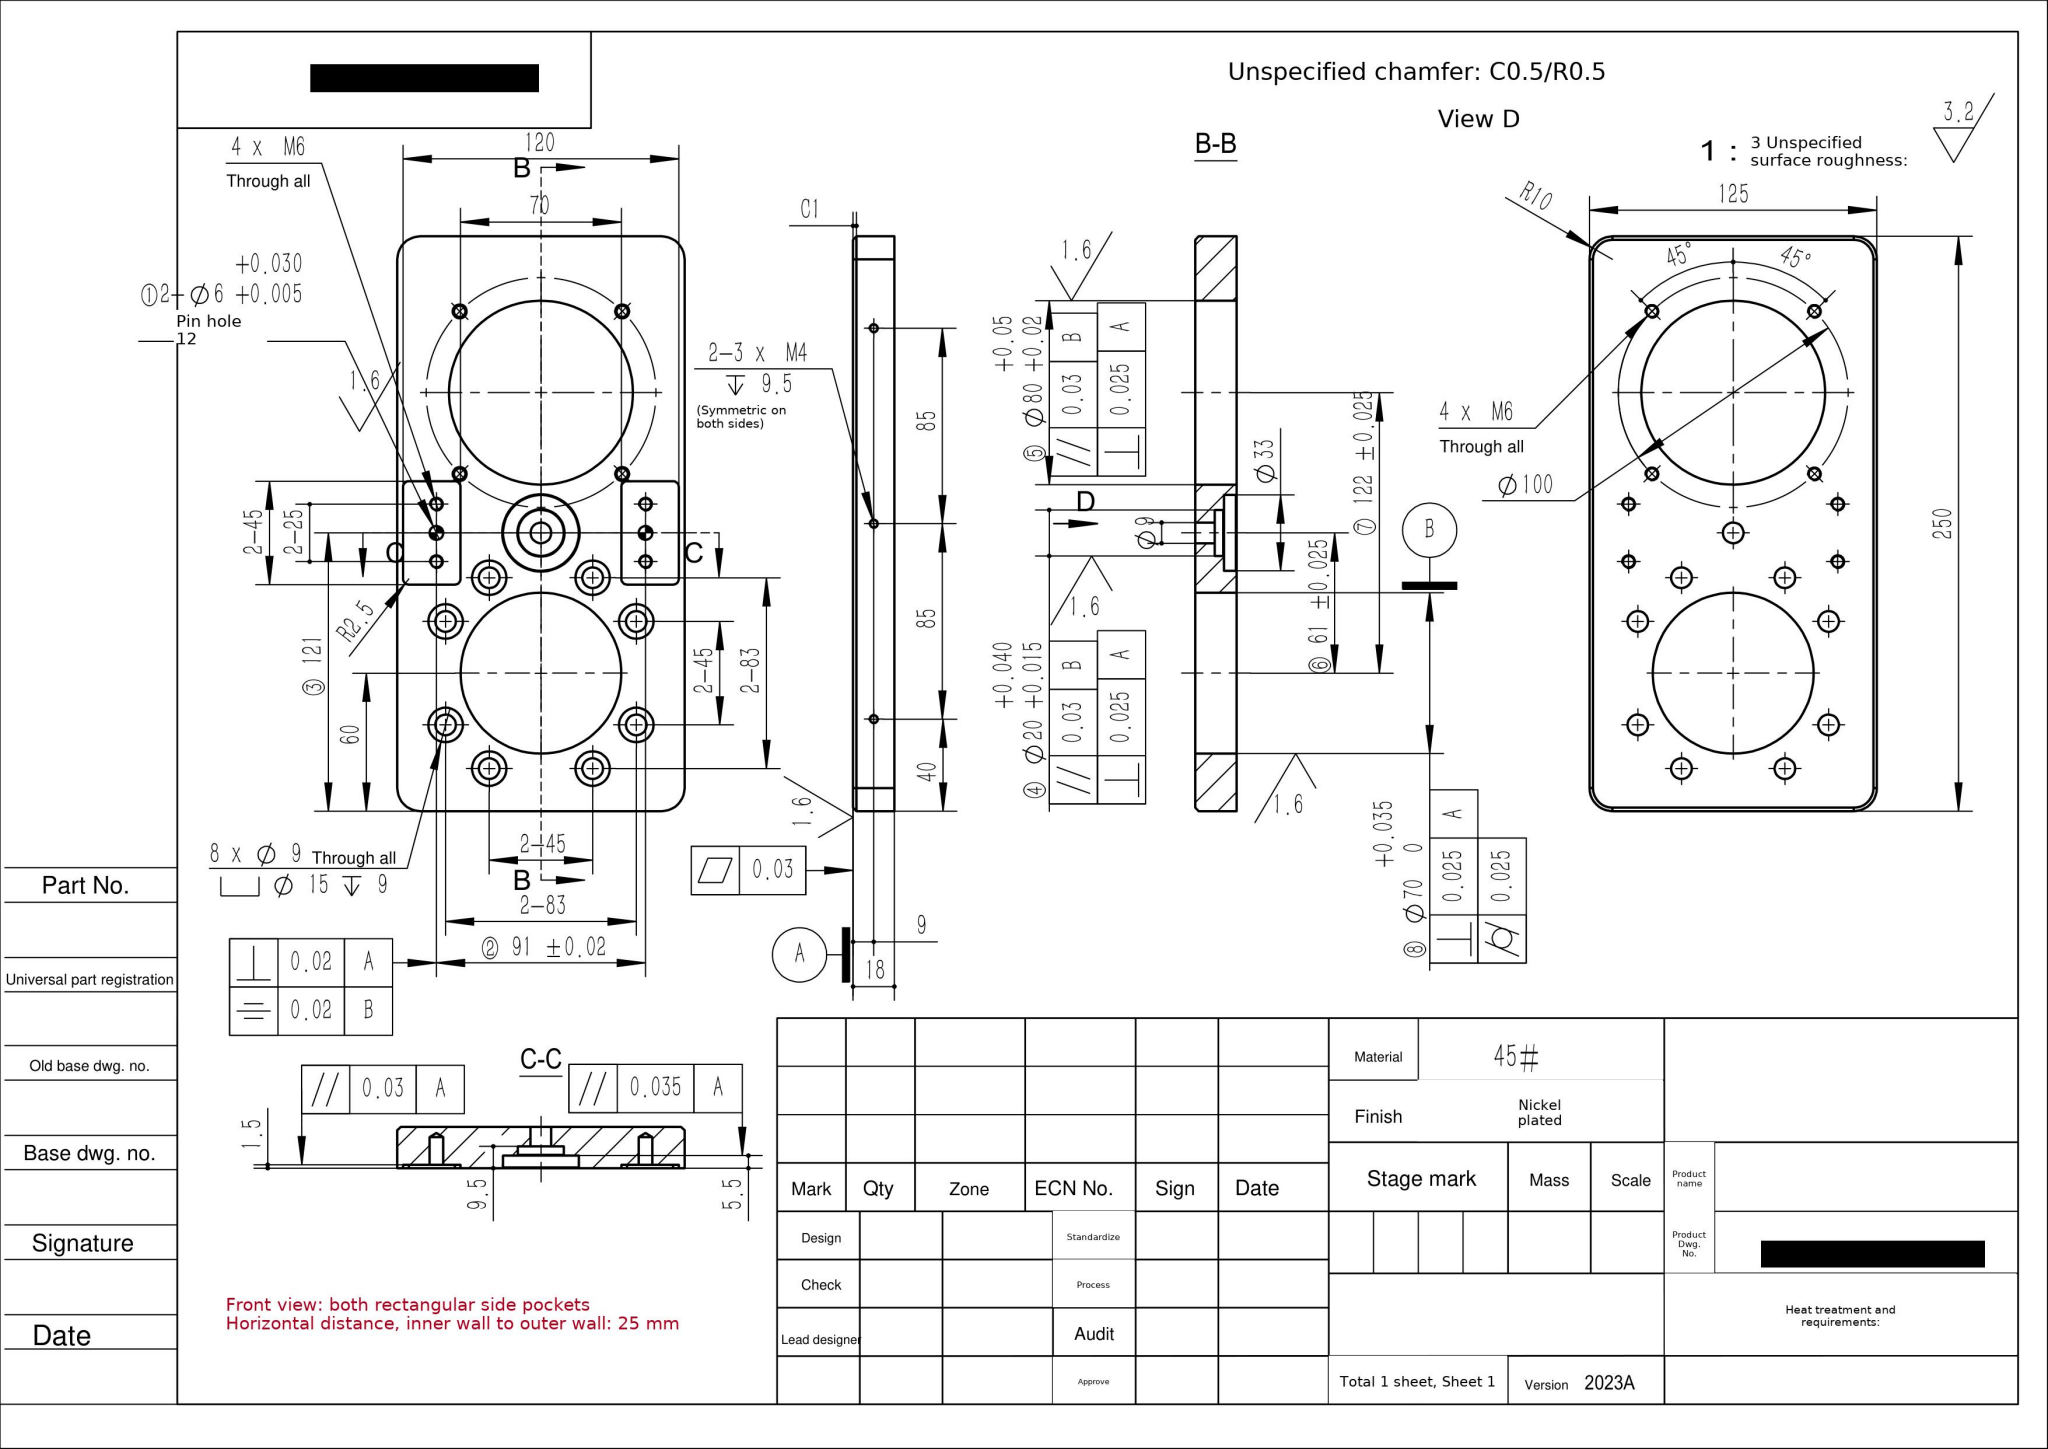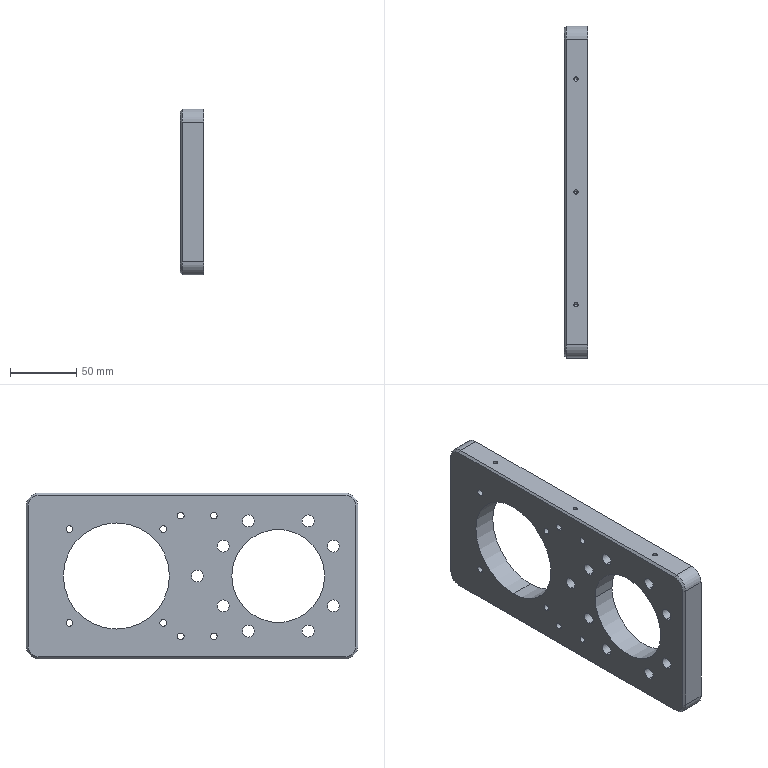Part | SolidWorks | mm | material 45# | 1 solid | 148 faces | box 18 x 250 x 125 mm | volume 369168 mm3 | cylinder 86 | cone 32 | plane 30 | commonest cylinder face diameters 5 x24 9 x18 15 x16 3.3 x12 20 x6 6 x4 33 x2 80 x2
build123d program:
from build123d import *

# Parameters (mm, degrees)
SKETCH1_W                                         = 250
SKETCH1_H                                         = 125
BOSS_EXTRUDE1_DEPTH                               = 18
SKETCH2_R                                         = 35
CUT_EXTRUDE1_DEPTH                                = 18
HOLE_SIZE_ACCORDING_TO_TYPE_12_OF_HEX_D           = 9
HOLE_SIZE_ACCORDING_TO_TYPE_12_OF_HEX_CBORE_D     = 15
HOLE_SIZE_ACCORDING_TO_TYPE_12_OF_HEX_CBORE_DEPTH = 9
MIRROR2_COPY_1_D                                  = 9
MIRROR2_COPY_1_CBORE_D                            = 15
MIRROR2_COPY_1_CBORE_DEPTH                        = 9
FILLET1_R                                         = 10
CHAMFER1_SIZE                                     = 1.5
SKETCH27_R                                        = 40
CUT_EXTRUDE7_DEPTH                                = 141.909
M6_TAPPED_HOLE1_D                                 = 5
M6_TAPPED_HOLE1_CSINK_D                           = 6.05
M6_TAPPED_HOLE1_CSINK_ANGLE                       = 90
CIRPATTERN1_COUNT                                 = 4
SKETCH31_R                                        = 16.5
CUT_EXTRUDE8_DEPTH                                = 5.5
SKETCH32_R                                        = 10
CUT_EXTRUDE9_DEPTH                                = 4
SKETCH33_R                                        = 4.5
CUT_EXTRUDE10_DEPTH                               = 141.077
CHAMFER2_SIZE                                     = 0.3
CUT_EXTRUDE11_DEPTH                               = 1.5
SIZE_MM_DOWEL_PIN_HOLE_1_D                        = 6
SIZE_MM_DOWEL_PIN_HOLE_1_DEPTH                    = 12
SIZE_MM_DOWEL_PIN_HOLE_1_TIP                      = 1.803
M6_TAPPED_HOLE2_D                                 = 5
M4_TAPPED_HOLE1_AT_2_COUNT                        = 2
M4_TAPPED_HOLE1_AT_2_PITCH                        = 85
M4_TAPPED_HOLE1_AT_3_COUNT                        = 2
M4_TAPPED_HOLE1_AT_3_PITCH                        = 170


with BuildPart() as part:
    # Sketch1 → Boss-Extrude1 (new body)
    with BuildSketch(Plane(origin=(0, 0, 0), x_dir=(0, -1, 0), z_dir=(1, 0, 0))):
        Rectangle(SKETCH1_W, SKETCH1_H)
    extrude(amount=BOSS_EXTRUDE1_DEPTH)

    # Sketch2 → Cut-Extrude1 (cut)
    with BuildSketch(Plane(origin=(18, 0, 0), x_dir=(0, -1, 0), z_dir=(1, 0, 0))):
        with Locations(Location((65, 0, 0), (0, 0, 180))):
            Circle(SKETCH2_R)
    extrude(amount=-CUT_EXTRUDE1_DEPTH, mode=Mode.SUBTRACT)

    # Hole Size _ according to_ Type 12 of Hex (through all)
    with Locations(Plane(origin=(18, 0, 0), x_dir=(0, -1, 0), z_dir=(1, 0, 0))):
        with Locations((106.5, 22.5), (87.5, 41.5)):
            hole_size_according_to_type_12_of_hex = CounterBoreHole(HOLE_SIZE_ACCORDING_TO_TYPE_12_OF_HEX_D / 2, HOLE_SIZE_ACCORDING_TO_TYPE_12_OF_HEX_CBORE_D / 2, HOLE_SIZE_ACCORDING_TO_TYPE_12_OF_HEX_CBORE_DEPTH)

    # Mirror1: Hole Size _ according to_ Type 12 of Hex across plane
    add(hole_size_according_to_type_12_of_hex.mirror(Plane.XY), mode=Mode.SUBTRACT)

    # Mirror2: Hole Size _ according to_ Type 12 of Hex across plane
    add(hole_size_according_to_type_12_of_hex.mirror(Plane(origin=(0, -65, 0), x_dir=(0, 0, 1), z_dir=(0, -1, 0))), mode=Mode.SUBTRACT)

    # Mirror2 copy 1 (through all)
    with Locations(Plane(origin=(18, -130, 0), x_dir=(0, 1, 0), z_dir=(1, 0, 0))):
        with Locations((106.5, 22.5), (87.5, 41.5)):
            CounterBoreHole(MIRROR2_COPY_1_D / 2, MIRROR2_COPY_1_CBORE_D / 2, MIRROR2_COPY_1_CBORE_DEPTH)

    # Fillet1
    fillet1_edges = [part.edges().sort_by_distance(p)[0] for p in [
        (9, -125, 62.5),
        (9, 125, 62.5),
        (9, 125, -62.5),
        (9, -125, -62.5),
    ]]
    fillet(fillet1_edges, radius=FILLET1_R)

    # Chamfer1
    chamfer1_edges = [part.edges().sort_by_distance(p)[0] for p in [
        (0, -125, 0),
        (0, 0, 62.5),
        (0, 125, 0),
        (0, 0, -62.5),
        (0, -122.071, -59.571),
        (0, 122.071, -59.571),
        (0, 122.071, 59.571),
        (0, -122.071, 59.571),
    ]]
    chamfer(chamfer1_edges, length=CHAMFER1_SIZE)

    # Sketch27 → Cut-Extrude7 (cut, through all)
    with BuildSketch(Plane(origin=(18, 0, 0), x_dir=(0, 0, -1), z_dir=(1, 0, 0))):
        with Locations((0, 57)):
            Circle(SKETCH27_R)
    extrude(amount=-CUT_EXTRUDE7_DEPTH, mode=Mode.SUBTRACT)

    # M6 Tapped Hole1 (through all)
    with Locations(Plane(origin=(18, 0, 0), x_dir=(0, 0, -1), z_dir=(1, 0, 0))):
        with Locations((35.355, 92.355)):
            m6_tapped_hole1 = CounterSinkHole(M6_TAPPED_HOLE1_D / 2, M6_TAPPED_HOLE1_CSINK_D / 2, counter_sink_angle=M6_TAPPED_HOLE1_CSINK_ANGLE)

    # CirPattern1: M6 Tapped Hole1 ×4 about axis
    cirpattern1_axis = Axis((0, 57, 0), (1, 0, 0))
    for i in range(1, CIRPATTERN1_COUNT):
        add(m6_tapped_hole1.rotate(cirpattern1_axis, i * 360 / CIRPATTERN1_COUNT), mode=Mode.SUBTRACT)

    # Sketch31 → Cut-Extrude8 (cut)
    with BuildSketch(Plane(origin=(18, 0, 0), x_dir=(0, 0, -1), z_dir=(1, 0, 0))):
        with Locations((0, -4)):
            Circle(SKETCH31_R)
    extrude(amount=-CUT_EXTRUDE8_DEPTH, mode=Mode.SUBTRACT)

    # Sketch32 → Cut-Extrude9 (cut)
    with BuildSketch(Plane(origin=(12.5, 0, 0), x_dir=(0, 0, -1), z_dir=(1, 0, 0))):
        with Locations((0, -4)):
            Circle(SKETCH32_R)
    extrude(amount=-CUT_EXTRUDE9_DEPTH, mode=Mode.SUBTRACT)

    # Sketch33 → Cut-Extrude10 (cut, through all)
    with BuildSketch(Plane(origin=(8.5, 0, 0), x_dir=(0, 0, -1), z_dir=(1, 0, 0))):
        with Locations((0, -4)):
            Circle(SKETCH33_R)
    extrude(amount=-CUT_EXTRUDE10_DEPTH, mode=Mode.SUBTRACT)

    # Chamfer2
    chamfer2_edges = [part.edges().sort_by_distance(p)[0] for p in [
        (18, -4, 16.5),
        (12.5, -4, 10),
    ]]
    chamfer(chamfer2_edges, length=CHAMFER2_SIZE)

    # Sketch34 → Cut-Extrude11 (cut)
    with BuildSketch(Plane(origin=(18, 0, 0), x_dir=(0, 0, -1), z_dir=(1, 0, 0))):
        with BuildLine():
            Line((37.5, 18.5), (57.5, 18.5))
            ThreePointArc((57.5, 18.5), (59.268, 17.768), (60, 16))
            Line((60, 16), (60, -24))
            ThreePointArc((60, -24), (59.268, -25.768), (57.5, -26.5))
            Line((57.5, -26.5), (37.5, -26.5))
            ThreePointArc((37.5, -26.5), (35.732, -25.768), (35, -24))
            Line((35, -24), (35, 16))
            ThreePointArc((35, 16), (35.732, 17.768), (37.5, 18.5))
        make_face()
    cut_extrude11 = extrude(amount=-CUT_EXTRUDE11_DEPTH, mode=Mode.SUBTRACT)

    # Mirror3: Cut-Extrude11 across plane
    add(cut_extrude11.mirror(Plane.XY), mode=Mode.SUBTRACT)

    # Size mm Dowel Pin Hole 1
    with Locations(Plane(origin=(16.5, 0, 0), x_dir=(0, 0, -1), z_dir=(1, 0, 0))):
        with Locations((45.5, -4), (-45.5, -4)):
            Hole(SIZE_MM_DOWEL_PIN_HOLE_1_D / 2, depth=SIZE_MM_DOWEL_PIN_HOLE_1_DEPTH)
            with Locations((0, 0, -(SIZE_MM_DOWEL_PIN_HOLE_1_DEPTH + SIZE_MM_DOWEL_PIN_HOLE_1_TIP / 2))):  # 118° drill point
                Cone(0, SIZE_MM_DOWEL_PIN_HOLE_1_D / 2, SIZE_MM_DOWEL_PIN_HOLE_1_TIP, mode=Mode.SUBTRACT)

    # M6 Tapped Hole2 (through all)
    with Locations(Plane(origin=(16.5, 0, 0), x_dir=(0, 0, -1), z_dir=(1, 0, 0))):
        with Locations((-45.5, 8.5), (-45.5, -16.5), (45.5, 8.5), (45.5, -16.5)):
            Hole(M6_TAPPED_HOLE2_D / 2)

    # Sketch44 → M4 Tapped Hole1 (revolve, cut)
    with BuildSketch(Plane(origin=(9, 85, -62.5), x_dir=(0, 1, 0), z_dir=(1, 0, 0))):
        Polygon((0, 0), (0, 12.591), (1.65, 11.6), (1.65, 0), align=None)
    m4_tapped_hole1 = revolve(axis=Axis((9, 85, -68.85), (0, 0, 1)), mode=Mode.SUBTRACT)

    # M4 Tapped Hole1 at 2: M4 Tapped Hole1 ×2
    with Locations(*[(0, -i * M4_TAPPED_HOLE1_AT_2_PITCH, 0) for i in range(1, M4_TAPPED_HOLE1_AT_2_COUNT)]):
        add(m4_tapped_hole1, mode=Mode.SUBTRACT)

    # M4 Tapped Hole1 at 3: M4 Tapped Hole1 ×2
    with Locations(*[(0, -i * M4_TAPPED_HOLE1_AT_3_PITCH, 0) for i in range(1, M4_TAPPED_HOLE1_AT_3_COUNT)]):
        add(m4_tapped_hole1, mode=Mode.SUBTRACT)

    # Mirror4: M4 Tapped Hole1 across plane
    add(m4_tapped_hole1.mirror(Plane.XY), mode=Mode.SUBTRACT)

    # Mirror4 copy 1 sketch → Mirror4 copy 1 (revolve, cut)
    with BuildSketch(Plane(origin=(9, 0, 62.5), x_dir=(0, 1, 0), z_dir=(1, 0, 0))):
        Polygon((0, 0), (0, -12.591), (1.65, -11.6), (1.65, 0), align=None)
    revolve(axis=Axis((9, 0, 68.85), (0, 0, 1)), mode=Mode.SUBTRACT)

    # Mirror4 copy 2 sketch → Mirror4 copy 2 (revolve, cut)
    with BuildSketch(Plane(origin=(9, -85, 62.5), x_dir=(0, 1, 0), z_dir=(1, 0, 0))):
        Polygon((0, 0), (0, -12.591), (1.65, -11.6), (1.65, 0), align=None)
    revolve(axis=Axis((9, -85, 68.85), (0, 0, 1)), mode=Mode.SUBTRACT)


solid = part.part